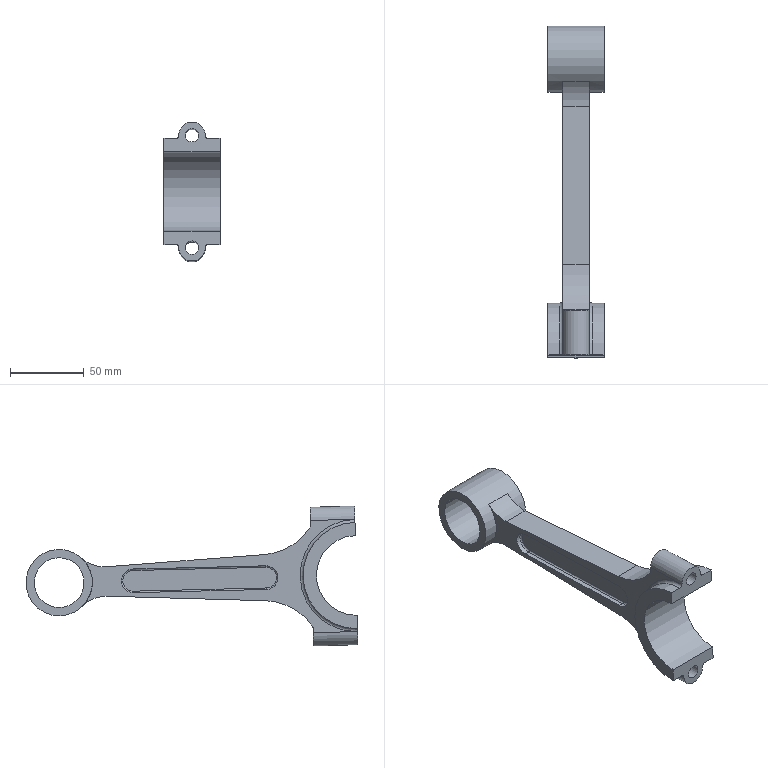Component | NX | 4_CONNECTING_ROD_3 | 1 solid | 49 faces | volume 133784 mm3 | cylinder 25 | plane 18 | torus 6 | commonest cylinder face diameters 6 x4 16 x4 2 x4 45 x3 80 x2 72 x2 18 x2 9 x2